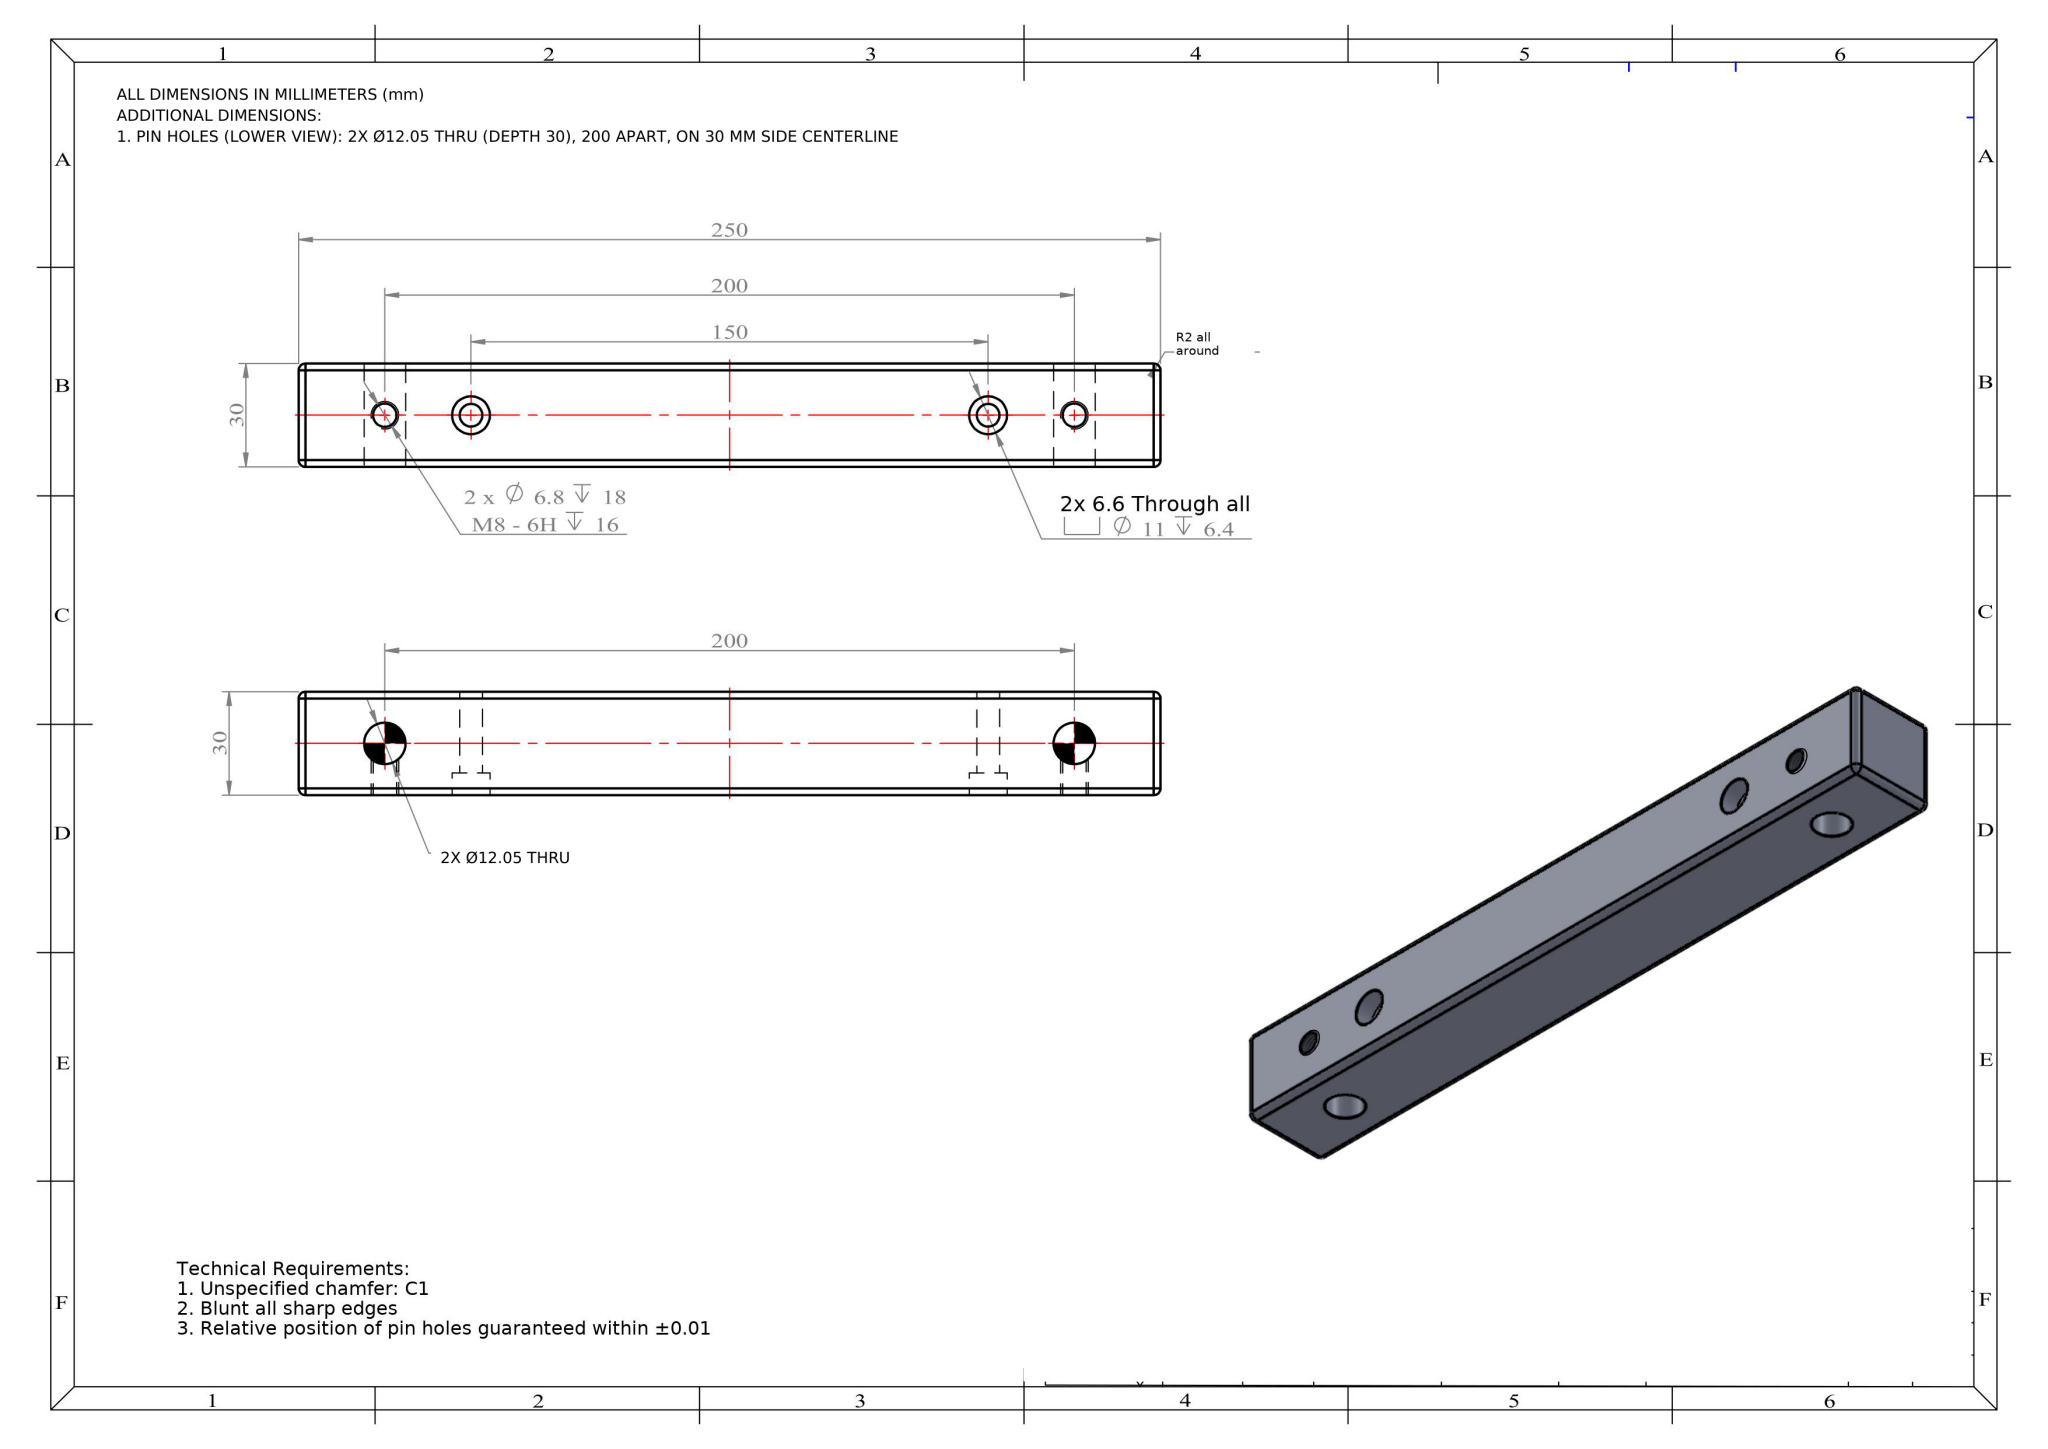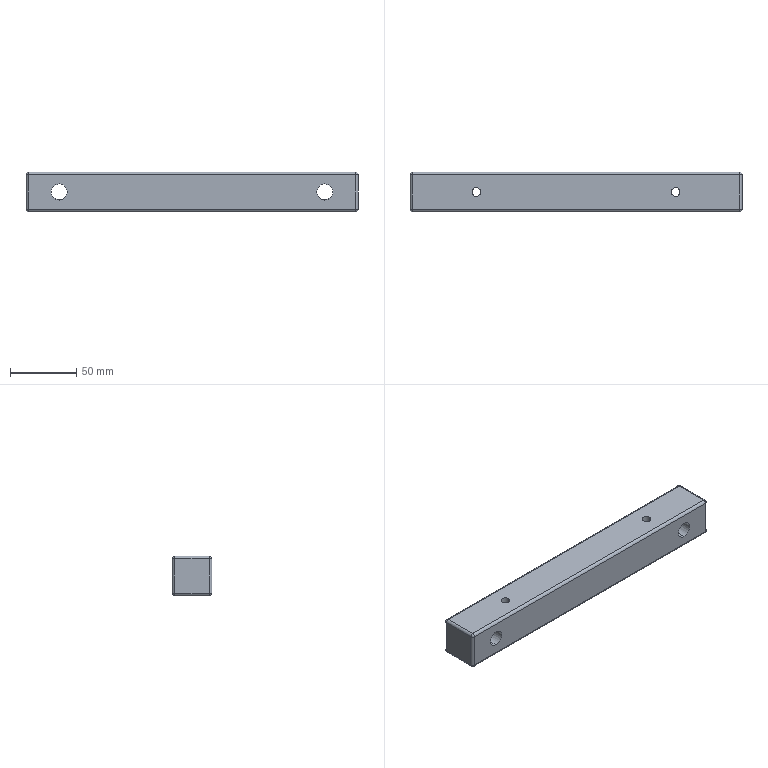Part | NX | mm | 1 solid | 44 faces | box 250 x 30 x 30 mm | volume 213602 mm3 | cylinder 28 | plane 8 | sphere 8 | commonest cylinder face diameters 4 x12 6.8 x4 12.05 x4 11 x4 6.6 x4